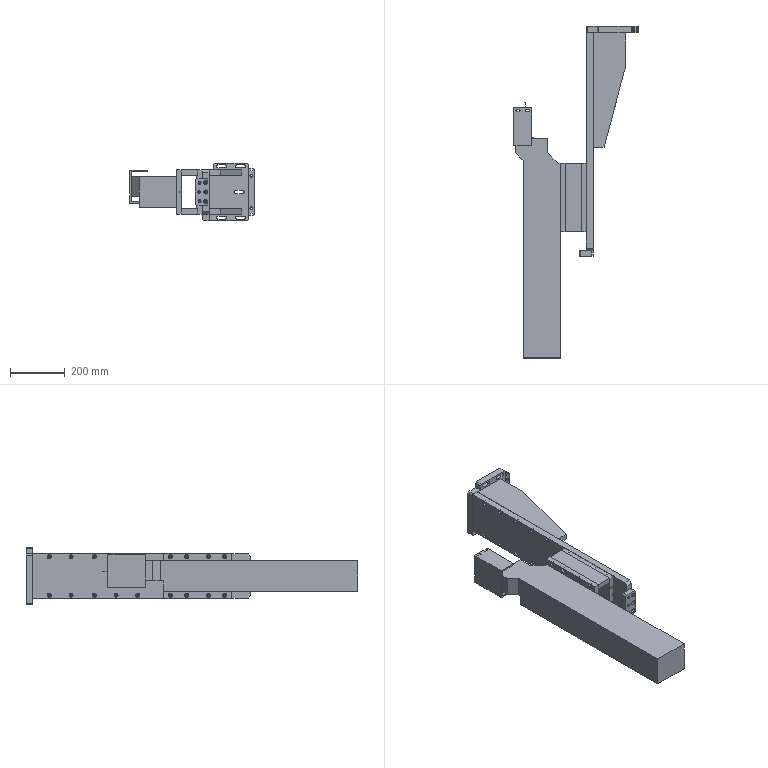Assembly | SolidWorks | mm | 12 component files | 12 solids | 685 faces | box 455.4 x 1217 x 212 mm | volume 19546126 mm3 | cylinder 383 | plane 220 | cone 82 | commonest cylinder face diameters 6.8 x84 15 x78 9 x78 11 x51 6 x32 6.6 x20 8.5 x20 5.5 x12
Bill of materials:
3120-HSC60-125 | 1 |  | Long rectangular bar with a stepped, narrower end section and a thin line-like protrusion from that end; one long side face has a pattern of small holes or points.
F1 | 1 |  | Narrow rectangular bar with a rectangular notch centered on each end, chamfered end corners, and a row of through holes on two faces.
F2 | 1 |  | Thick plate with a stepped (notched) corner outline, chamfered corners, and many round holes and elongated slots, plus a small hole in one edge.
F3 | 2 |  | Flat plate with a constant thickness whose outline tapers along its length, with one straight edge and one angled edge, ending in a wider rectangular section.
F4 | 1 |  | Long flat bar with one chamfered end, two rows of three elongated slots and two single holes near that end, two rows of five small holes along the long edges, and three holes in the end face.
F5 | 1 |  | Thick rectangular block with chamfered corners and six through holes in two columns of three, with mixed hole sizes.
F6 | 1 |  | Rectangular plate with a long groove running along its face, a raised or stepped region on one face, holes in a grid on the face, and holes in the edges.
F7 | 2 |  | Plain rectangular block with a row of four evenly spaced holes in one long side face.
F8 | 1 |  | Rectangular plate with a shallow raised pad or step on one face, holes around the perimeter, and inner holes in columns and a center row.
F9 | 1 |  | Thin, uniform-thickness channel (U-shaped) bracket: two parallel flanges joined by a web, with two elongated slots near the free edge of each flange.
Mates:
1. coincident | 3120-HSC60-125-1 face at (0, 113.279, 0) dir (0, 0, 1) | assembly plane at (0, 0, 0) dir (0, 0, 1)
2. coincident | 3120-HSC60-125-1 face at (0, 113.279, 0) dir (1, 0, 0) | assembly plane at (0, 0, 0) dir (1, 0, 0)
3. width | 3120-HSC60-125-1 face at (-46.473, 203.279, -74) dir (0, 0, -1) | 3120-HSC60-125-1 face at (0, 113.279, 0) dir (0, 0, 1) | F9-1 face at (-164.4, 317.279, -92) dir (0, 0, 1) | F9-1 face at (-164.4, 317.279, 18) dir (0, 0, -1)
4. coincident | 3120-HSC60-125-1 face at (-164.4, 203.279, 0) dir (-1, 0, 0) | F9-1 face at (-164.4, 317.279, 18) dir (1, 0, 0)
5. coincident | F8-1 face at (18, 113.279, 25) dir (1, 0, 0) | F7-2 face at (18, 113.279, 5) dir (-1, 0, 0)
6. coincident | F8-1 face at (20, -156.721, 25) dir (0, 0, 1) | F7-2 face at (78, -136.721, 25) dir (0, 0, 1)
7. coincident | F8-1 face at (20, -136.721, -137) dir (0, -1, 0) | F7-2 face at (78, -136.721, 5) dir (0, -1, 0)
8. coincident | F4-4 face at (121, 594.279, -137) dir (1, 0, 0) | F3-1 face at (121, 172.279, -137) dir (-1, 0, 0)
9. coincident | F4-4 face at (121, -206.721, -137) dir (0, 0, -1) | F3-1 face at (121, 172.279, -137) dir (0, 0, -1)
10. coincident | F4-4 face at (121, -206.721, 25) dir (0, 0, 1) | F3-2 face at (121, 172.279, 25) dir (0, 0, 1)
11. coincident | F4-4 face at (121, 594.279, -137) dir (1, 0, 0) | F3-2 face at (121, 172.279, 5) dir (-1, 0, 0)
12. distance | F6-1 face at (96, -136.721, -137) dir (0, -1, 0) | F4-4 face at (121, -206.721, -137) dir (0, -1, 0)
13. coincident | F4-4 face at (121, -206.721, -137) dir (0, -1, 0) | F5-1 face at (71, -206.721, -6) dir (0, 1, 0)
14. width | F4-4 face at (121, -206.721, 25) dir (0, 0, 1) | F4-4 face at (121, -206.721, -137) dir (0, 0, -1) | F5-1 face at (121, -226.721, -106) dir (0, 0, -1) | F5-1 face at (121, -226.721, -6) dir (0, 0, 1)
15. coincident | F4-4 face at (121, 594.279, -137) dir (1, 0, 0) | F5-1 face at (121, -226.721, -6) dir (1, 0, 0)
16. coincident | F8-1 face at (18, 113.279, -137) dir (1, 0, 0) | F7-1 face at (18, 113.279, -137) dir (-1, 0, 0)
17. coincident | F8-1 face at (20, 113.279, -117) dir (0, 0, -1) | F7-1 face at (78, -136.721, -117) dir (0, 0, 1)
18. coincident | F8-1 face at (20, -136.721, -137) dir (0, -1, 0) | F7-1 face at (78, -136.721, -137) dir (0, -1, 0)
19. coincident | F7-1 face at (78, 113.279, -137) dir (1, 0, 0) | F6-1 face at (78, 113.279, -137) dir (-1, 0, 0)
20. coincident | F7-1 face at (78, -136.721, -117) dir (0, 0, 1) | F6-1 face at (76, 113.279, -117) dir (0, 0, -1)
21. coincident | F7-1 face at (78, -136.721, -137) dir (0, -1, 0) | F6-1 face at (96, -136.721, -137) dir (0, -1, 0)
22. coincident | F6-1 face at (96, 113.279, -137) dir (1, 0, 0) | F4-4 face at (96, 594.279, -137) dir (-1, 0, 0)
23. coincident | F4-4 face at (121, 594.279, -137) dir (0, 1, 0) | F2-1 face at (96, 594.279, 50) dir (0, -1, 0)
24. coincident | F4-4 face at (121, 594.279, -137) dir (1, 0, 0) | F2-1 face at (121, 592.279, 50) dir (-1, 0, 0)
25. width | F2-1 face at (96, 617.279, -162) dir (0, 0, -1) | F2-1 face at (96, 617.279, 50) dir (0, 0, 1) | F4-4 face at (121, -206.721, 25) dir (0, 0, 1) | F4-4 face at (121, -206.721, -137) dir (0, 0, -1)
26. coincident | F1-1 face at (266, 617.279, 29) dir (0, 1, 0) | F2-1 face at (96, 617.279, 50) dir (0, 1, 0)
27. width | F2-1 face at (96, 617.279, 50) dir (0, 0, 1) | F2-1 face at (96, 617.279, -162) dir (0, 0, -1) | F1-1 face at (266, 592.279, -141) dir (0, 0, -1) | F1-1 face at (266, 592.279, 29) dir (0, 0, 1)
28. coincident | F1-1 face at (266, 592.279, -141) dir (-1, 0, 0) | F2-1 face at (266, 617.279, -162) dir (1, 0, 0)
29. distance | F9-1 face at (-104.4, 178.279, 23) dir (0, -1, 0) | 3120-HSC60-125-1 face at (-164.4, 203.279, 0) dir (0, 1, 0)